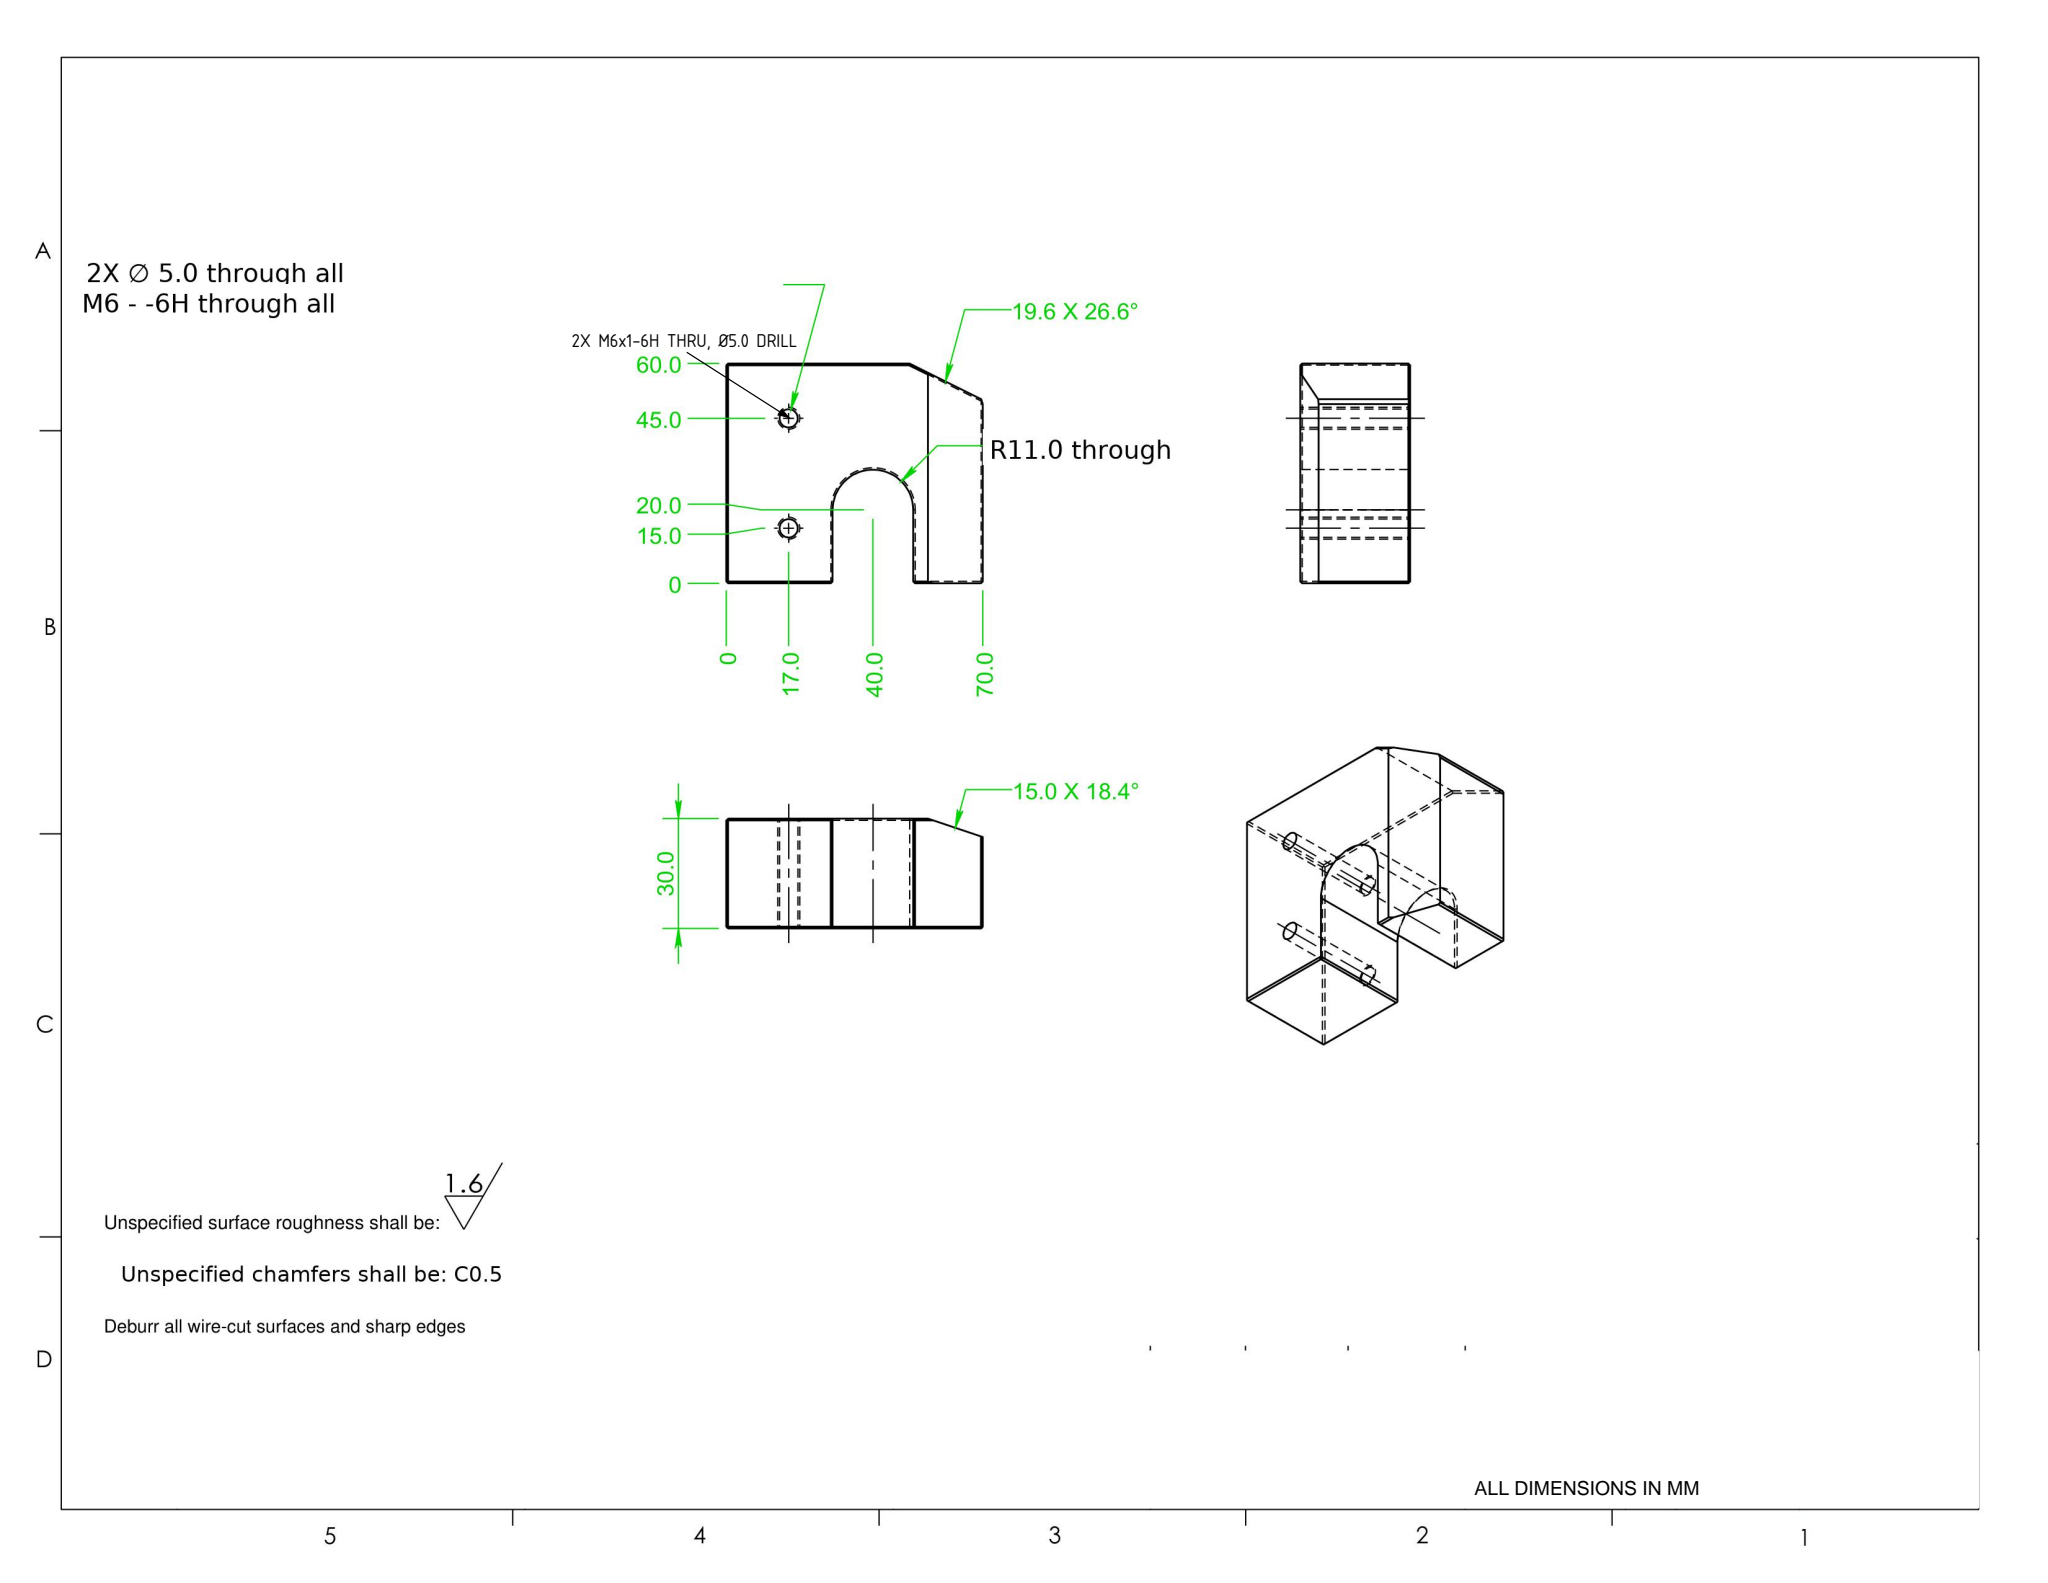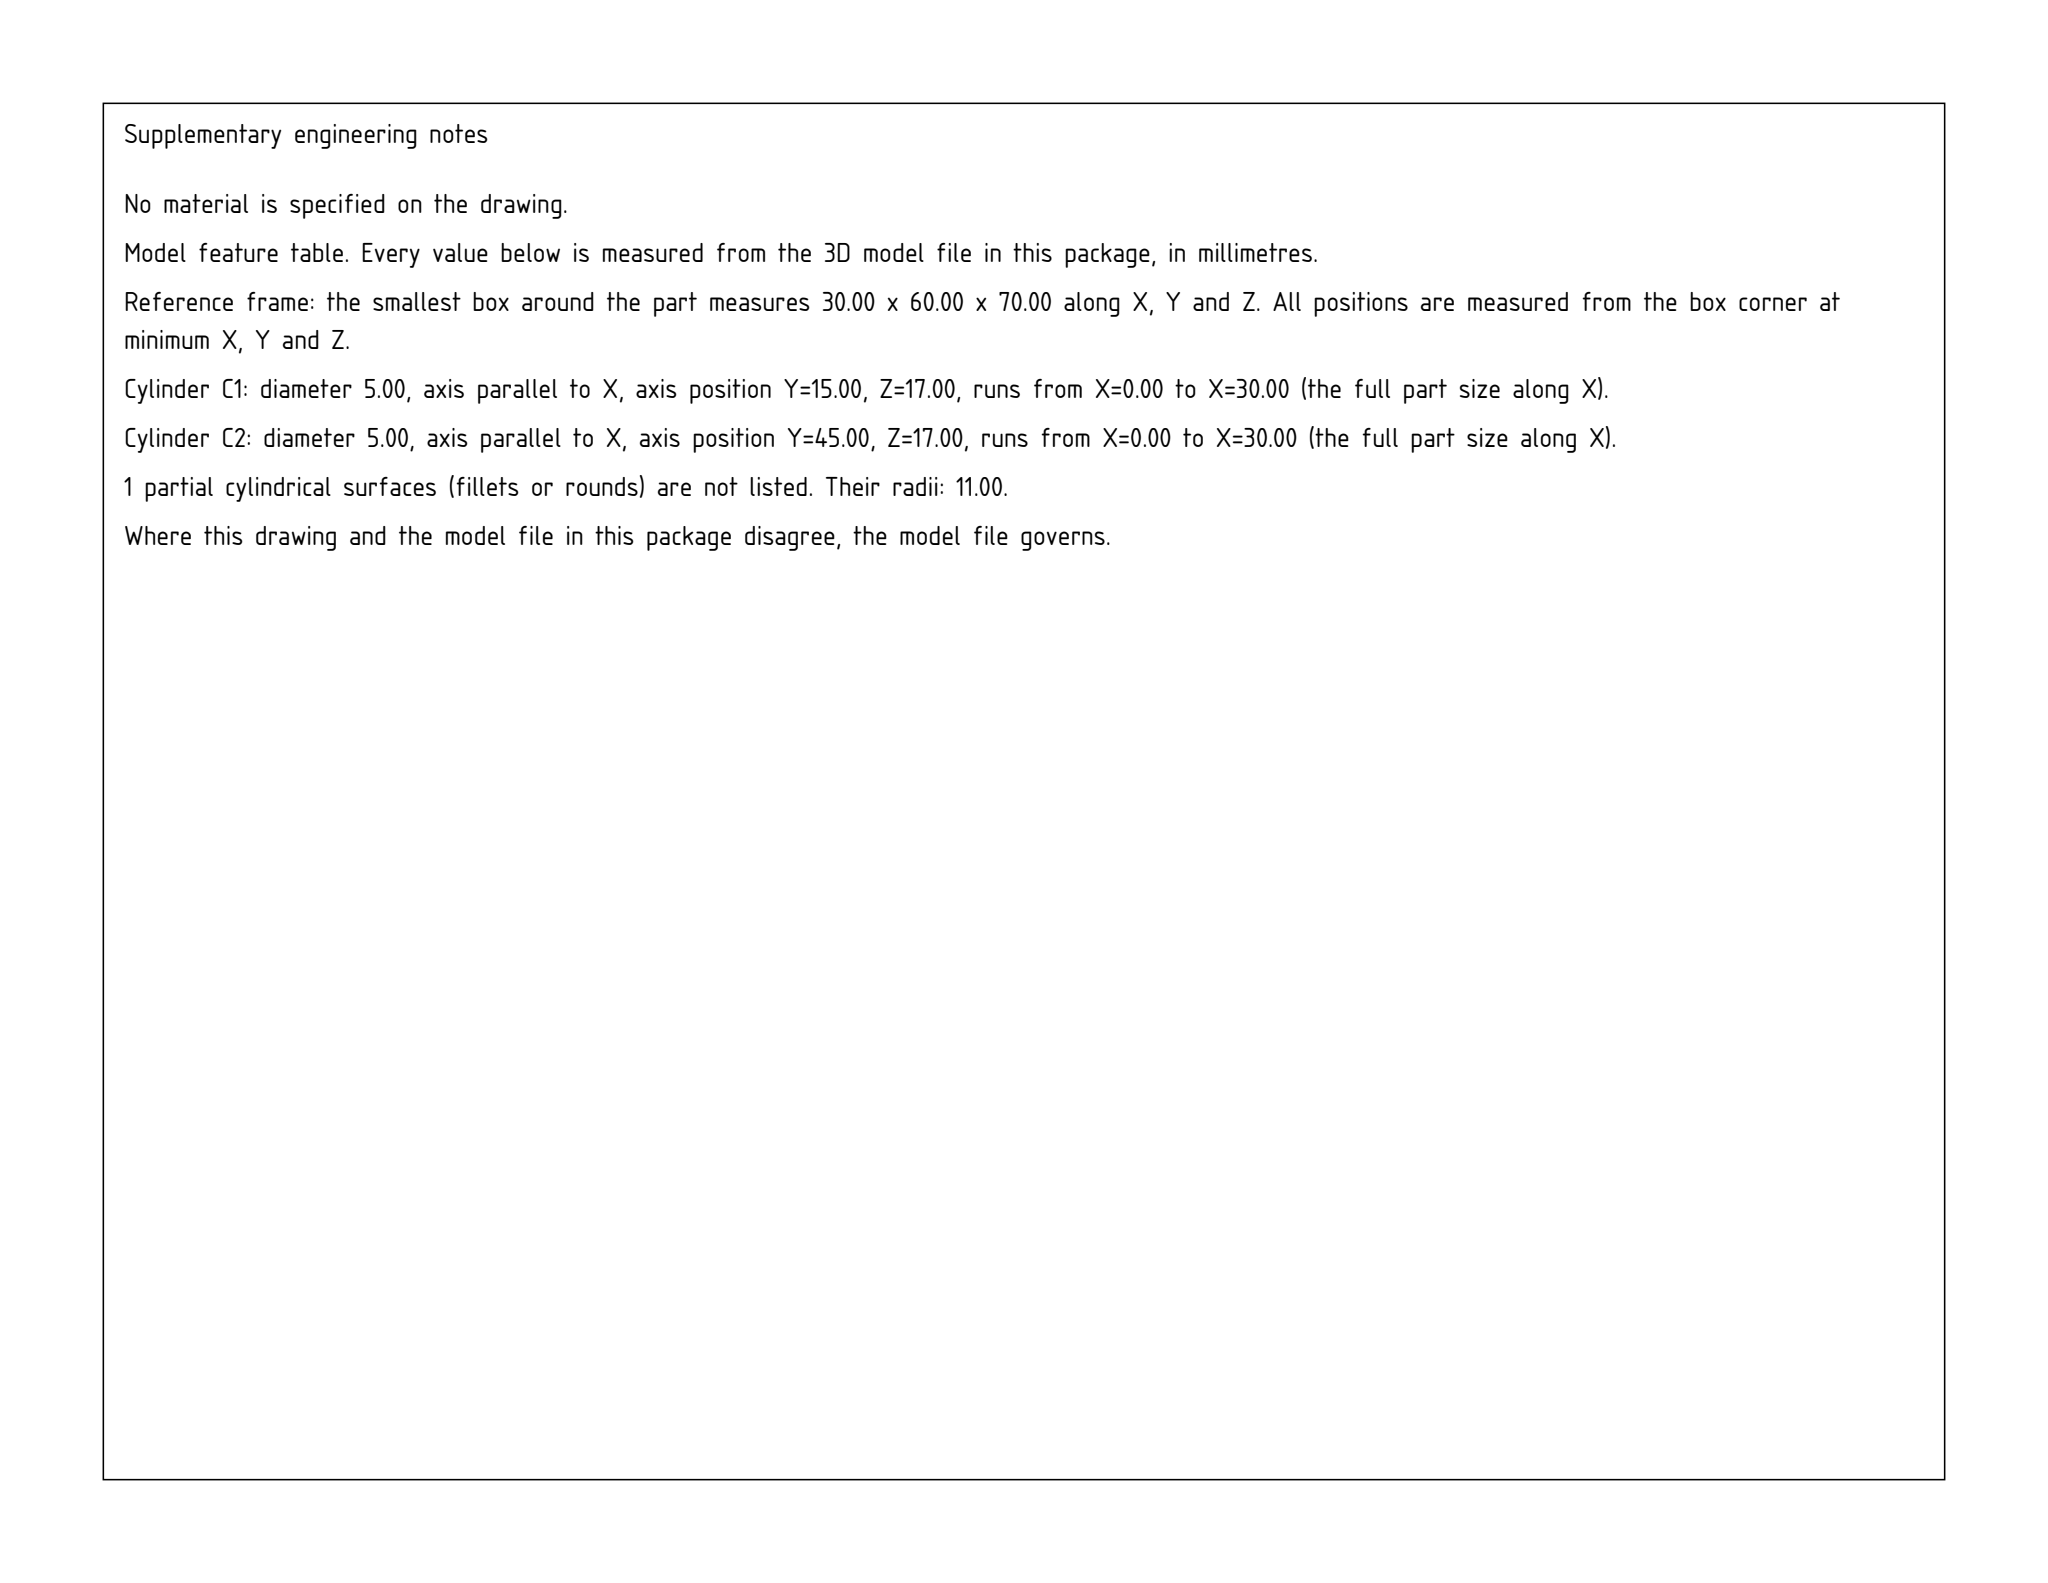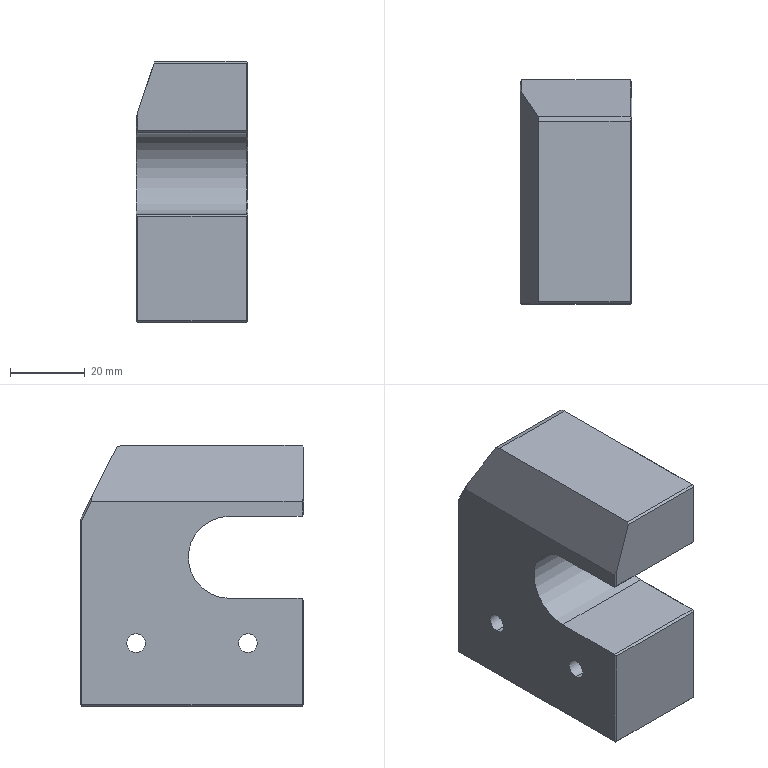Part | SolidWorks | mm | 1 solid | 36 faces | box 30 x 60 x 70 mm | volume 100871 mm3 | plane 30 | cylinder 5 | cone 1 | commonest cylinder face diameters 5 x4 22 x1
Drawing notes:
2X M6x1 - 6H THRU ALL, TAP DRILL Ø5.0 THRU | from the solid: Two Ø5.0 x 30.0 holes on X axis at (y15,z17) and (y45,z17); Ø5.0 = M6x1 tap drill